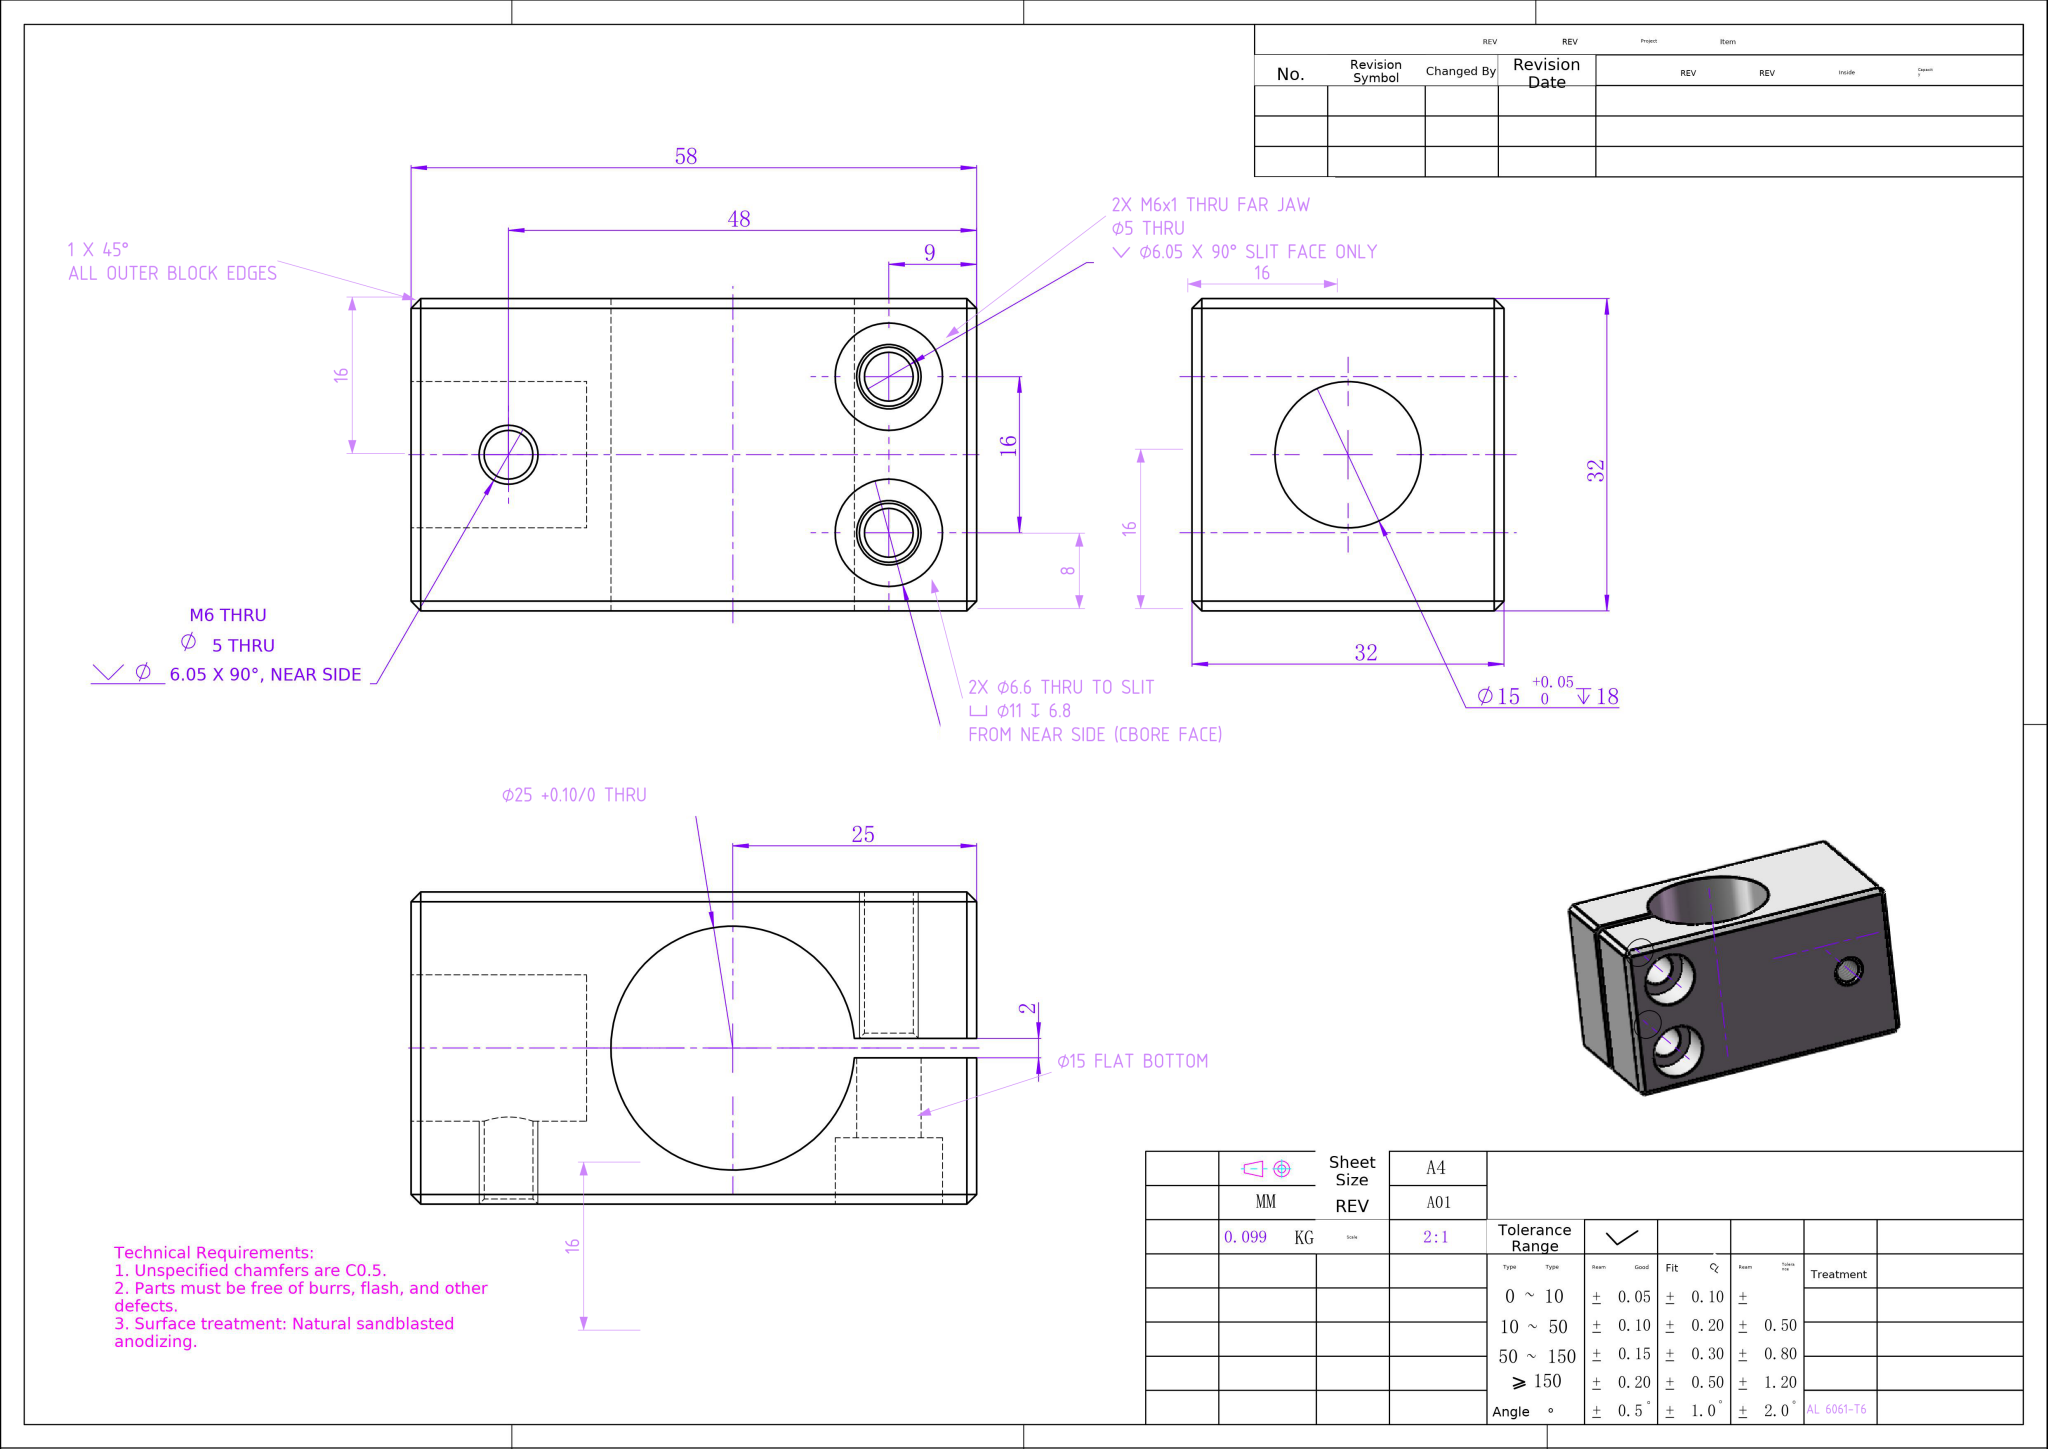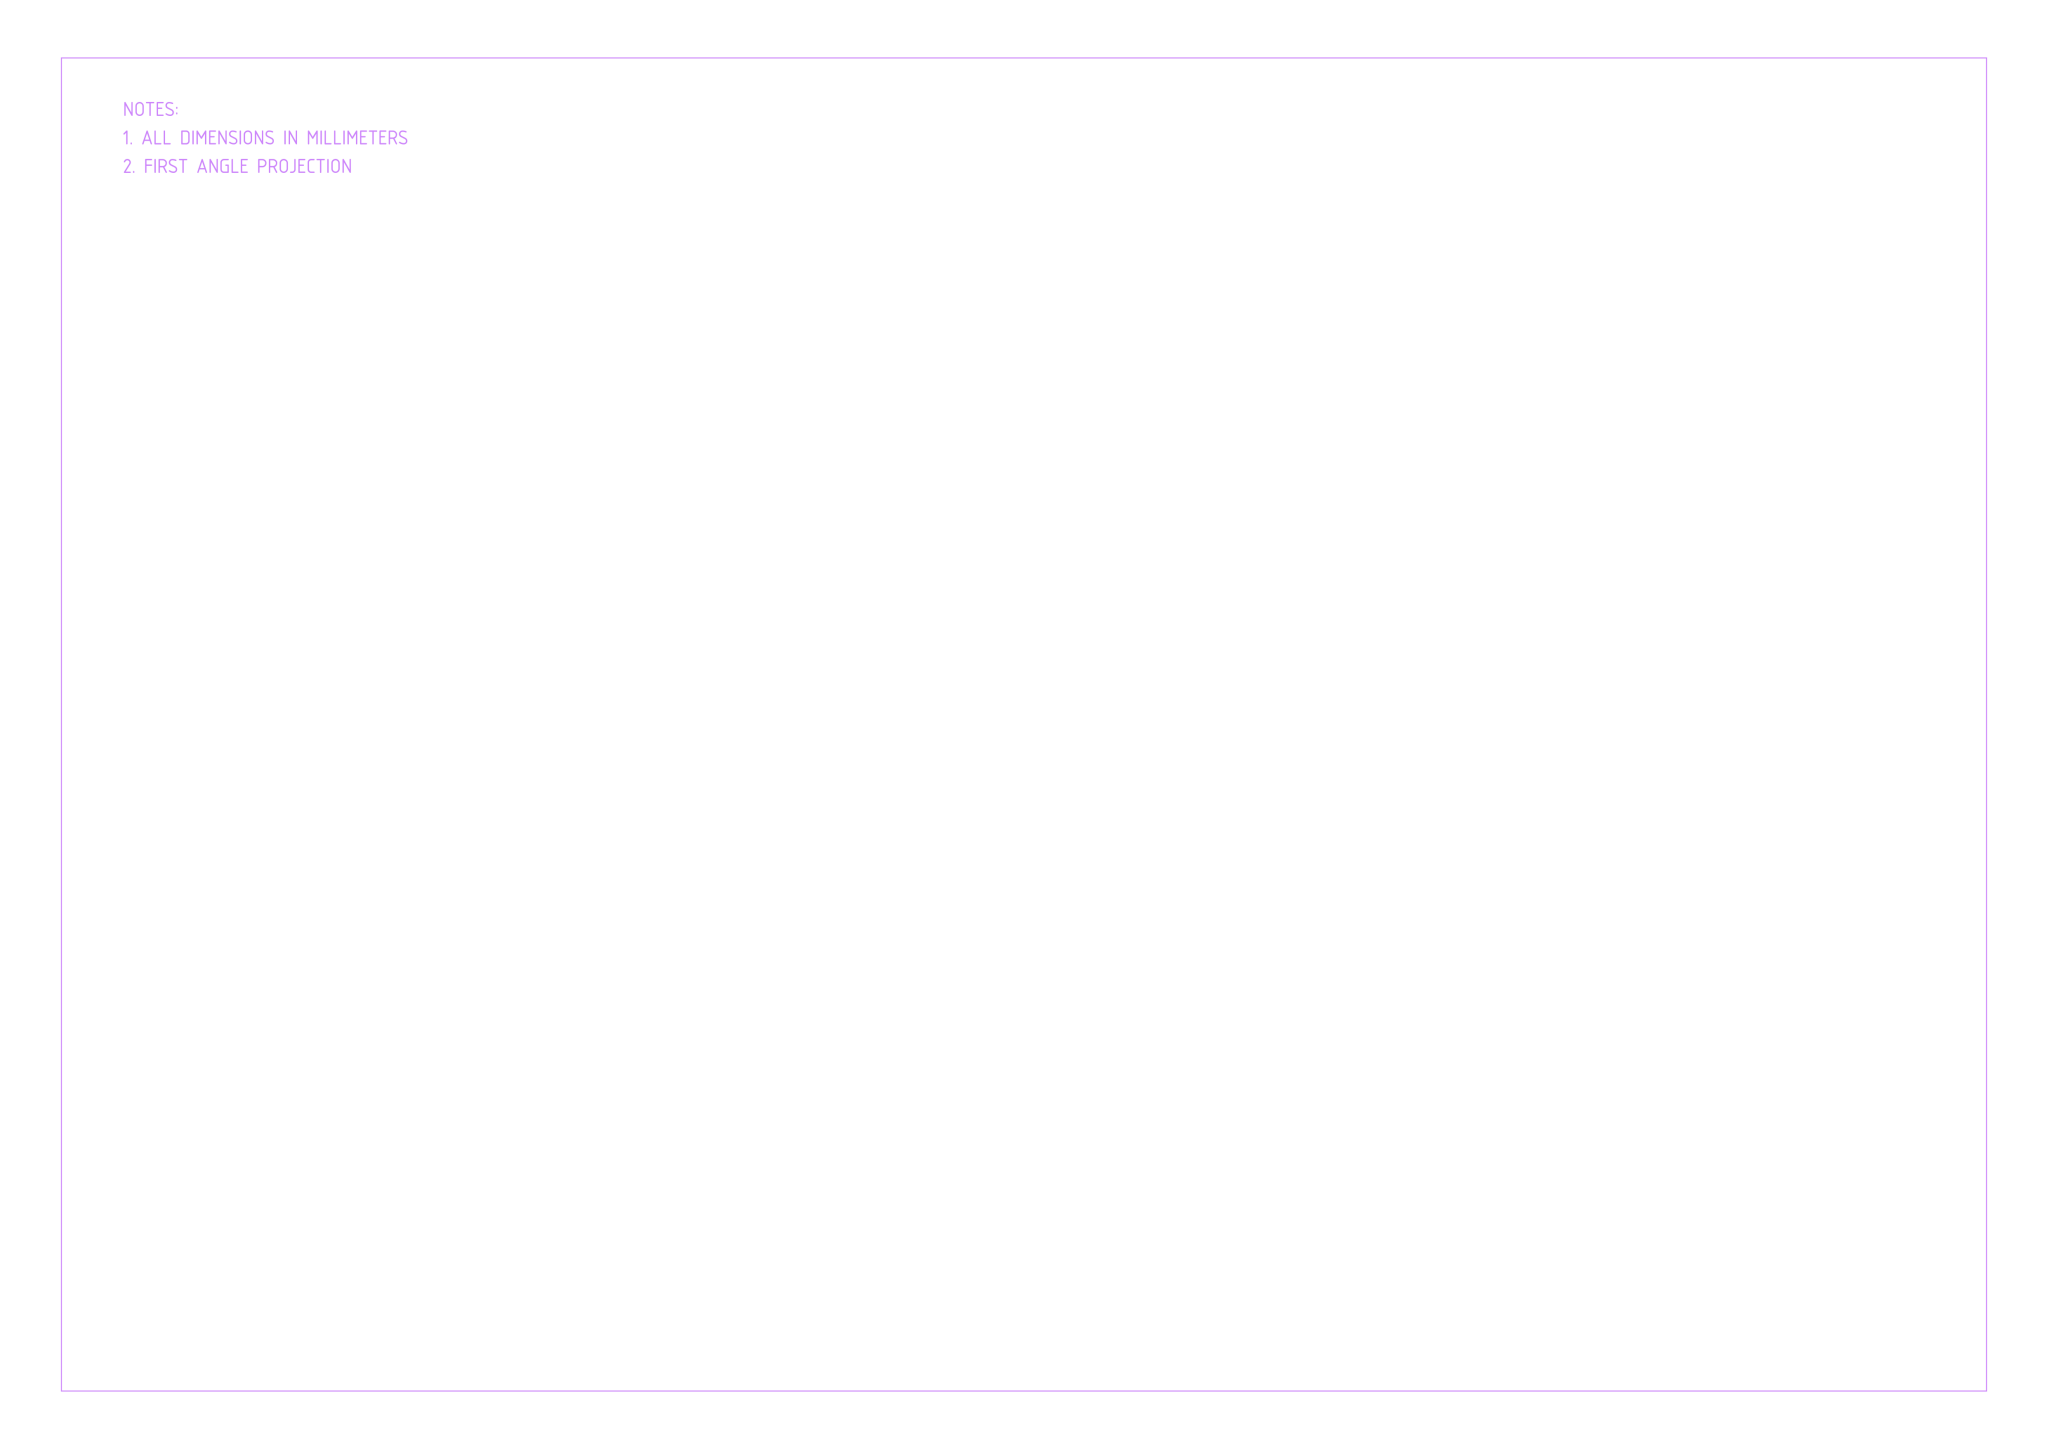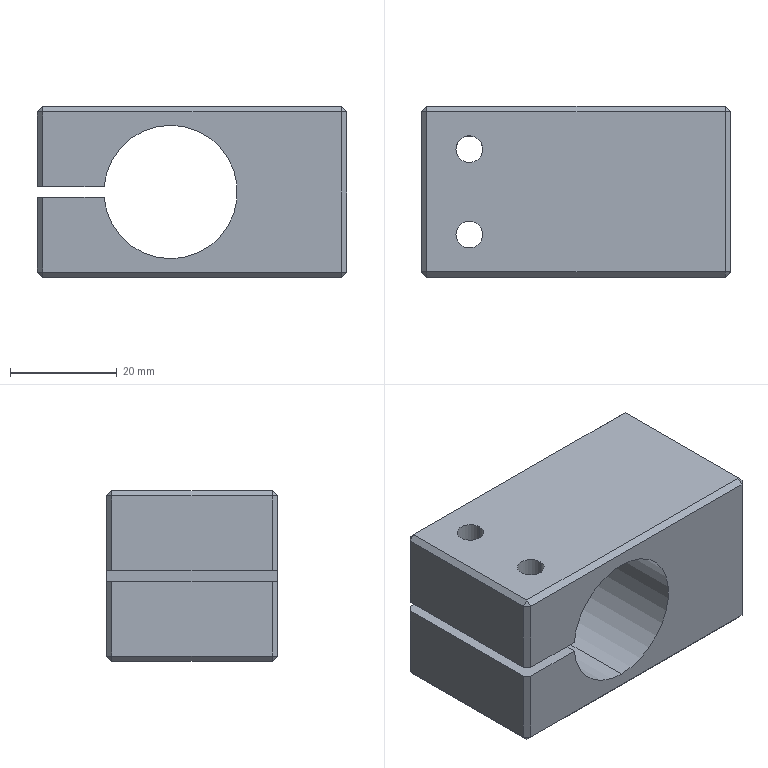Part | NX | mm | Dual-Port Stepped Manifold Block | 1 solid | 59 faces | box 58 x 32 x 32 mm | volume 36847 mm3 | plane 34 | cylinder 19 | cone 6 | commonest cylinder face diameters 5 x6 6.6 x4 11 x4 25 x3 15 x2